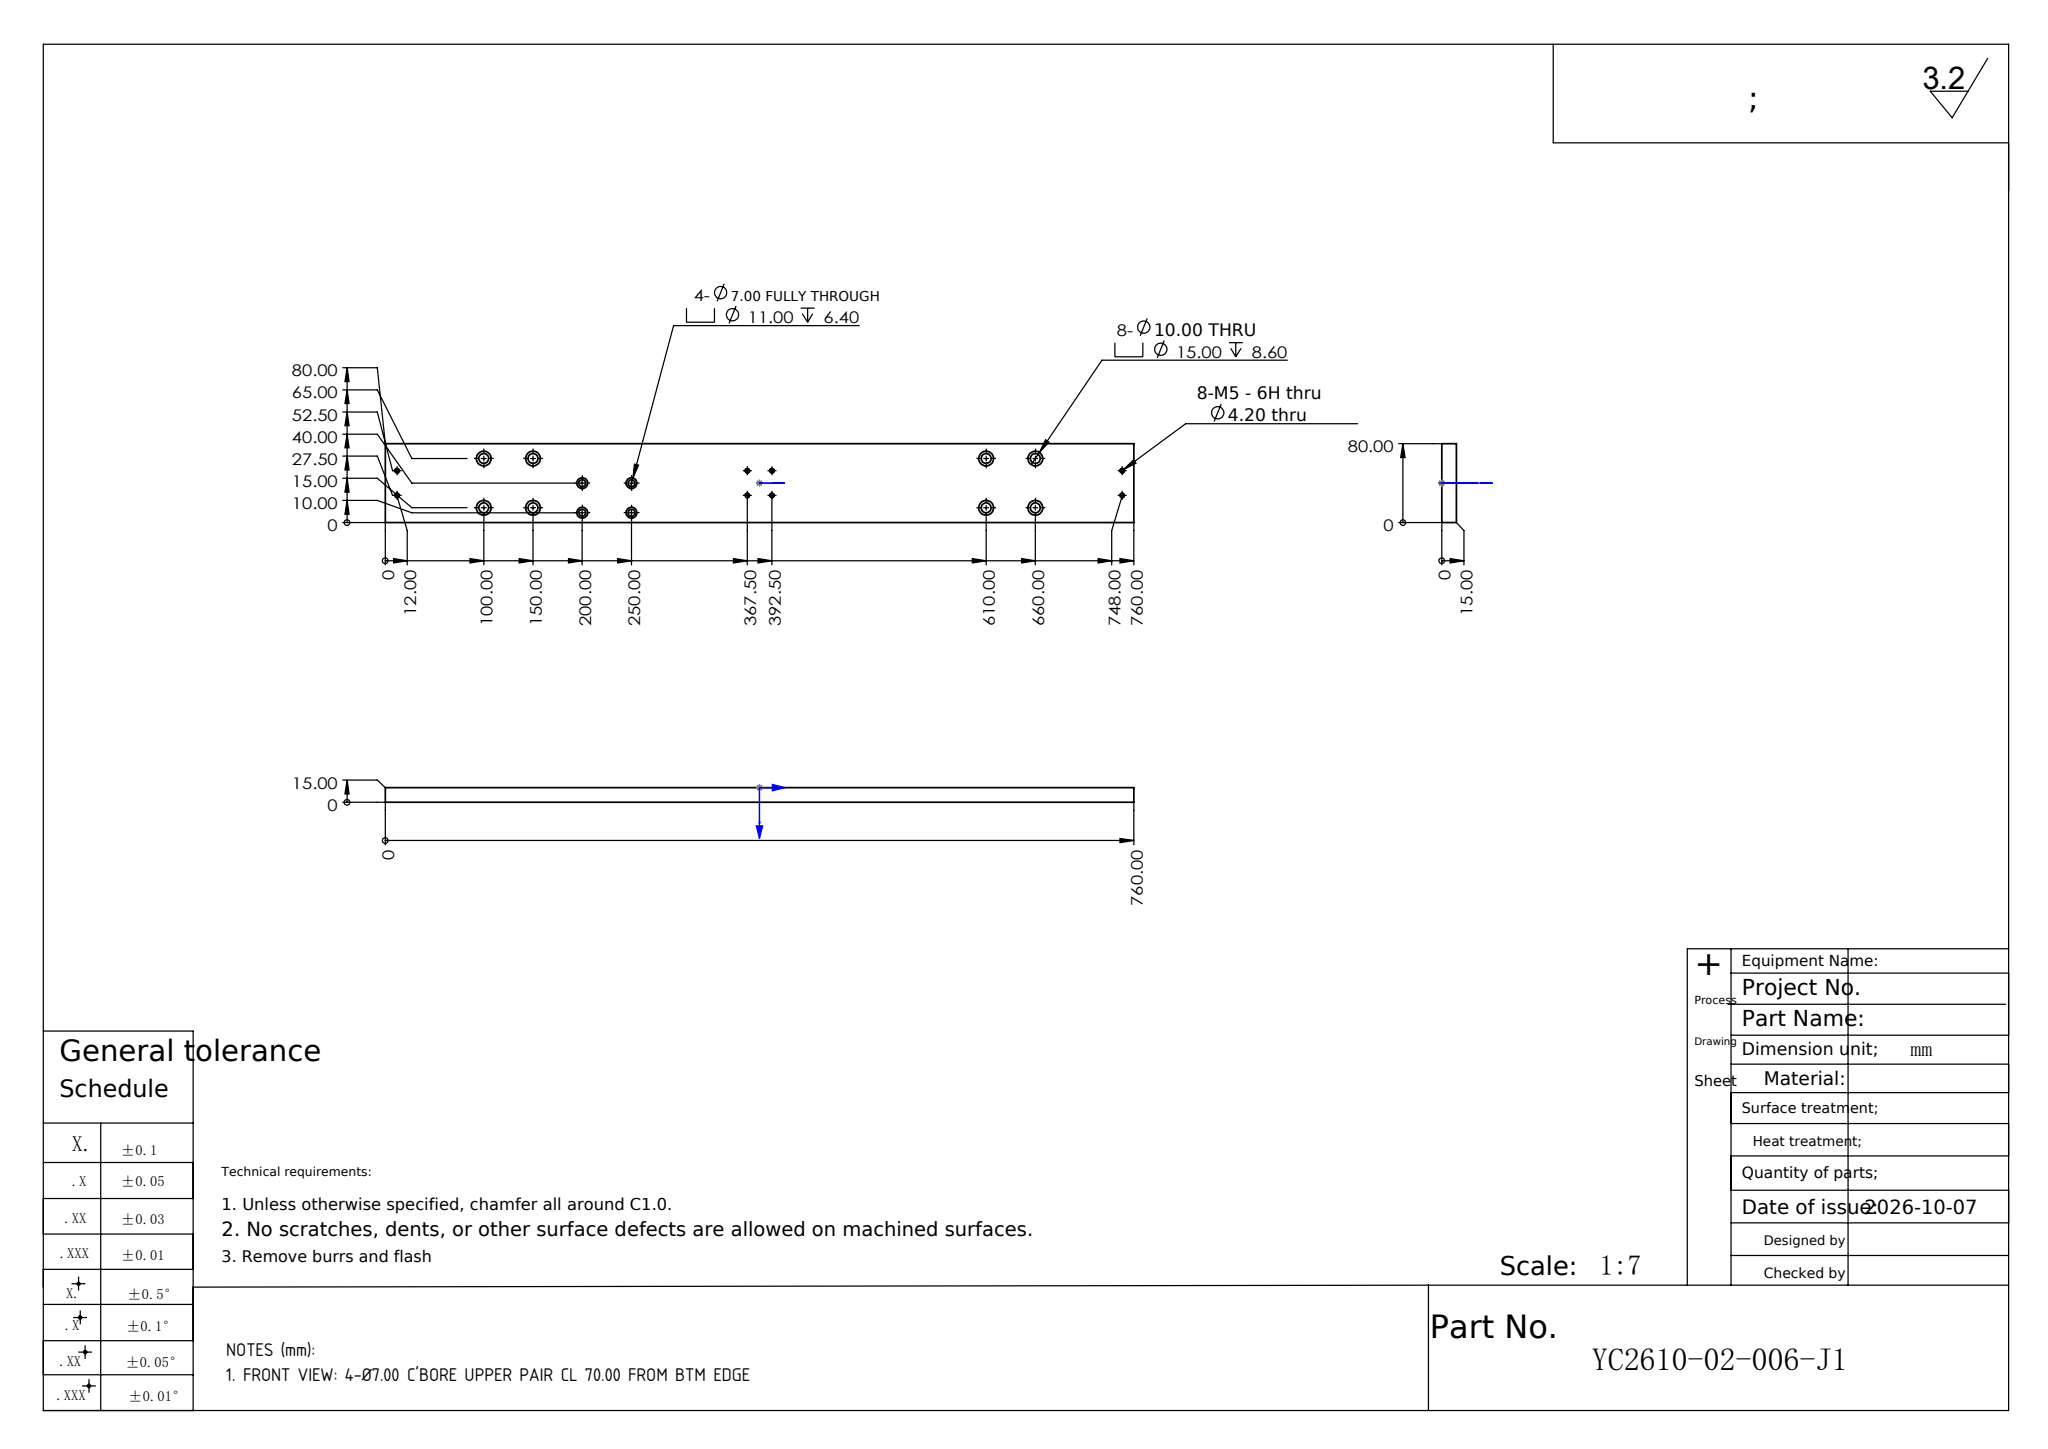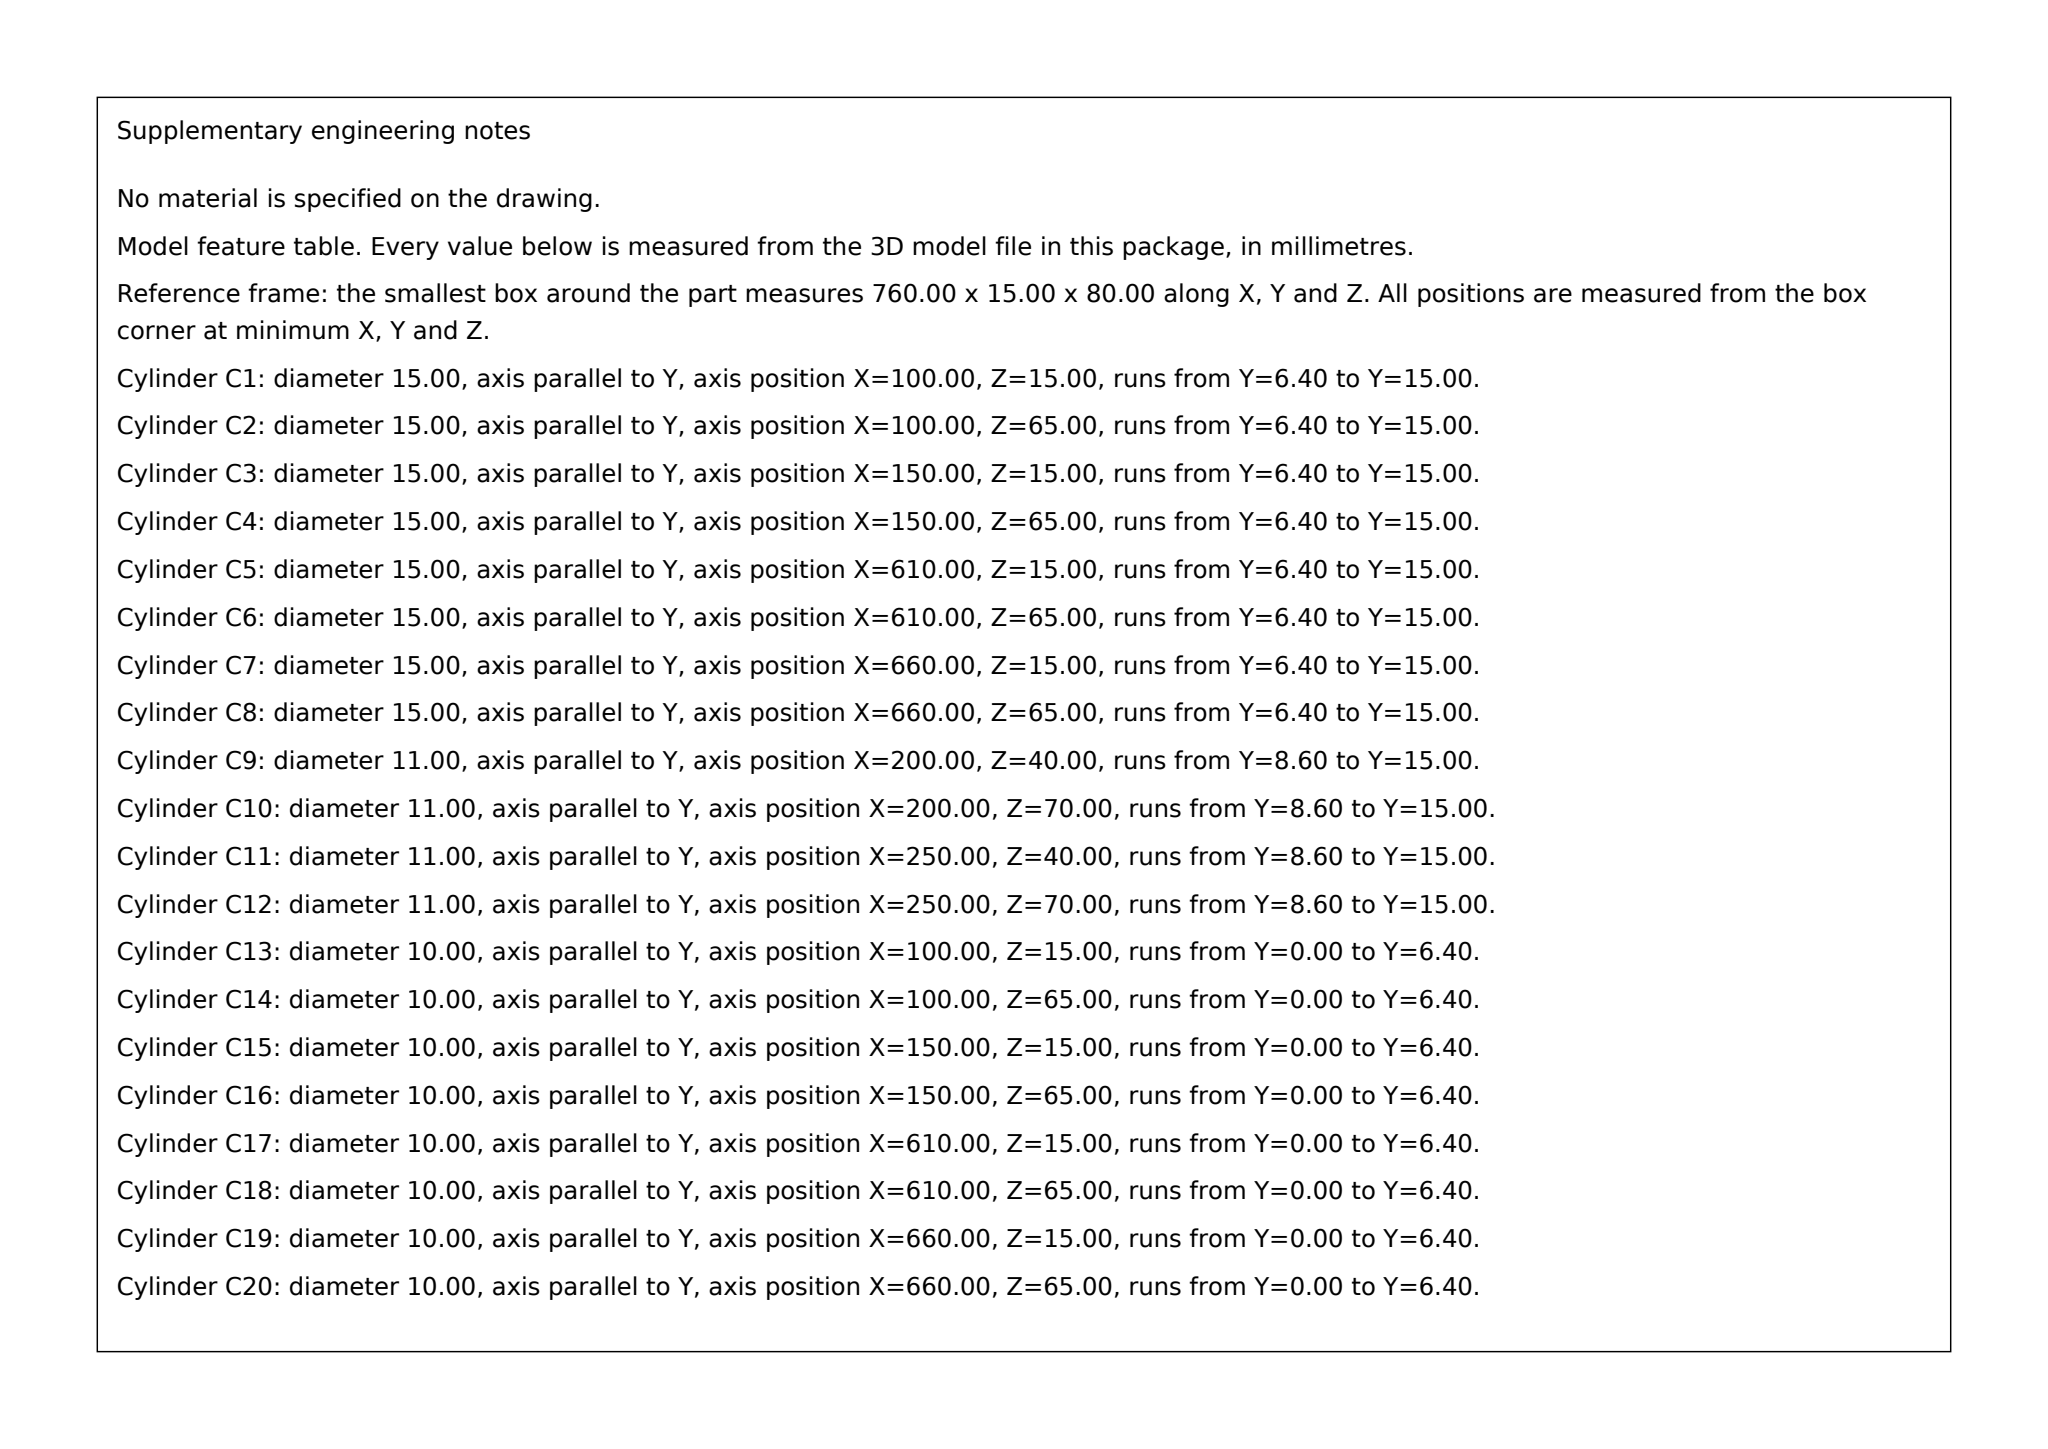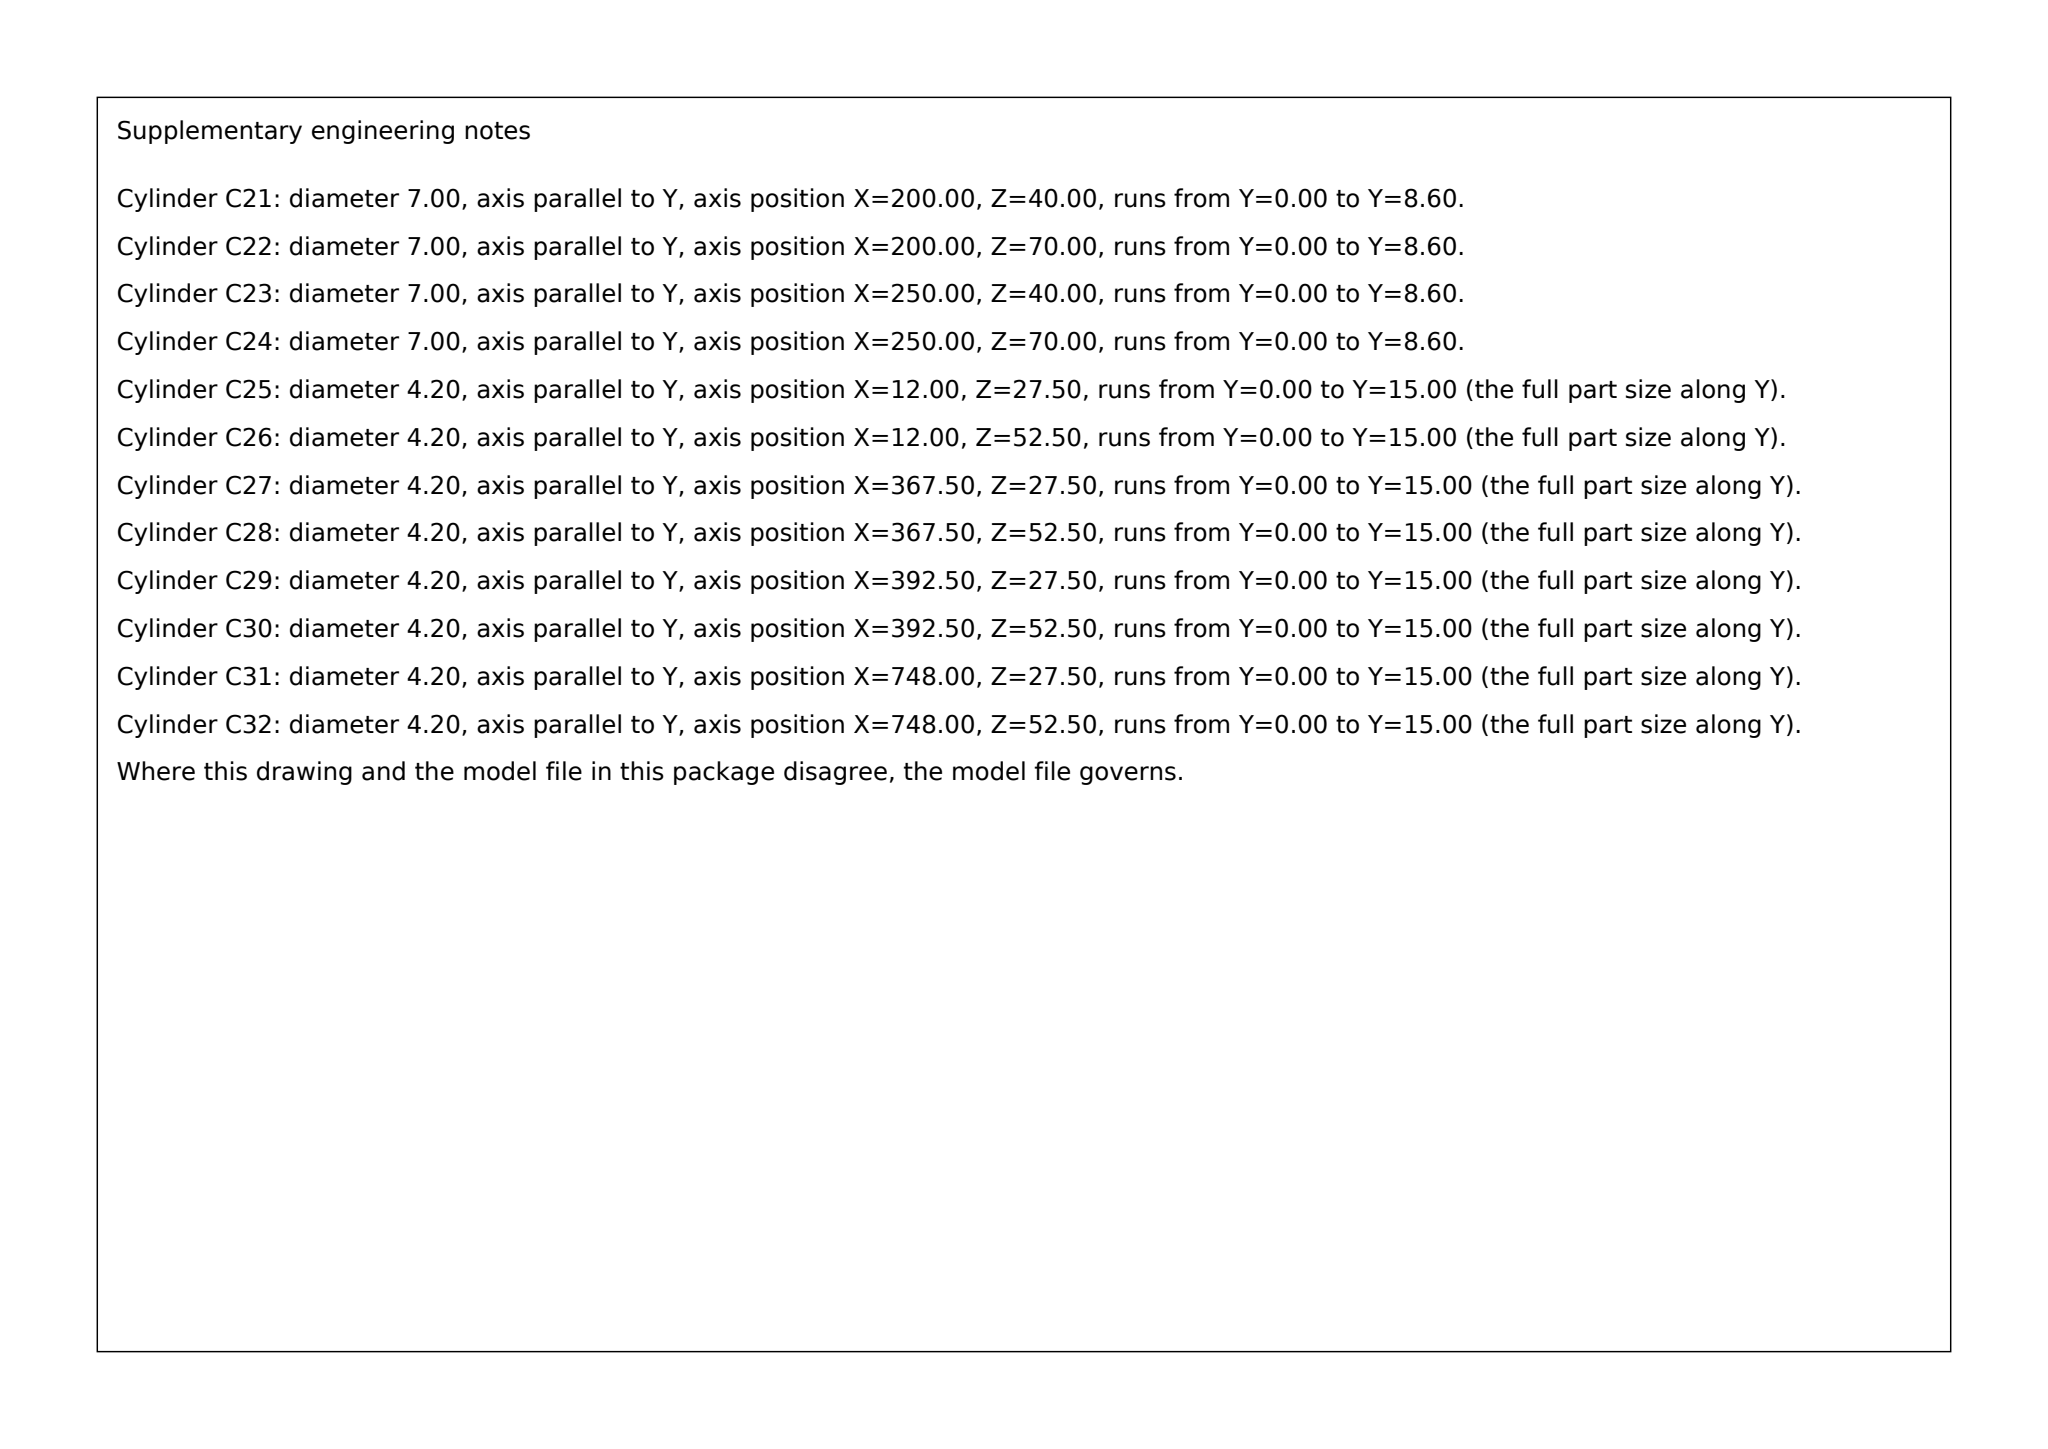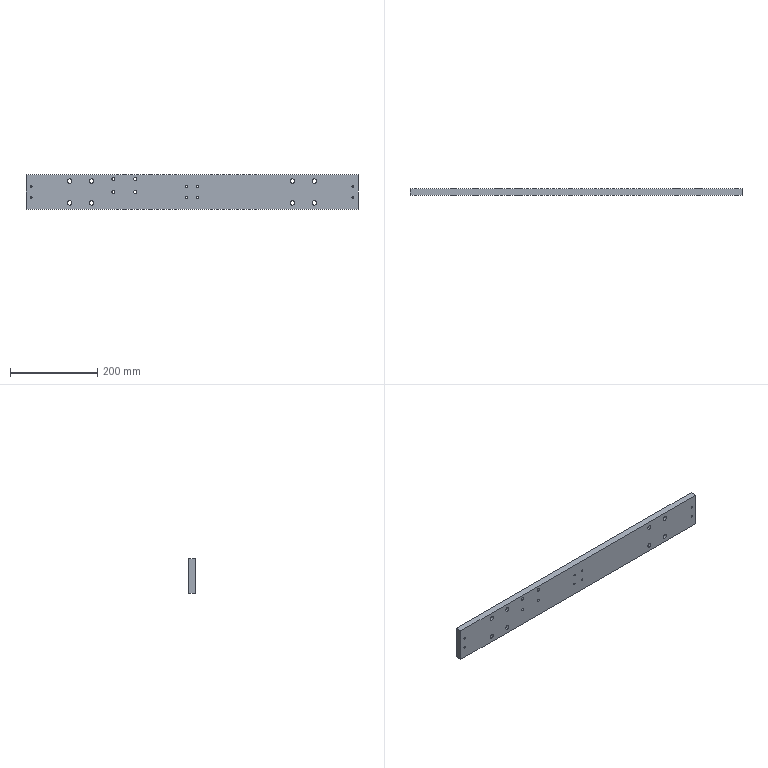Part | SolidWorks | mm | 1 solid | 82 faces | box 760 x 15 x 80 mm | volume 890402 mm3 | cylinder 64 | plane 18 | commonest cylinder face diameters 15 x16 10 x16 4.2 x16 11 x8 7 x8
Drawing notes:
FRONT VIEW: 4-Ø7.00 C'BORE UPPER PAIR CL 70.00 FROM BTM EDGE | from the solid: Ø7.0/Ø11.0 cyls at (x=200,z=70) and (x=250,z=70); bbox z=0..80
build123d program:
from build123d import *

# Parameters (mm, degrees)
SKETCH1_W                                       = 760
SKETCH1_H                                       = 80
BOSS_EXTRUDE1_DEPTH                             = 15
M5_TAPPED_HOLE1_D                               = 4.2
M6_HEX_SOCKET_HEAD_CAP_SCREW_CBORE1_D           = 7
M6_HEX_SOCKET_HEAD_CAP_SCREW_CBORE1_CBORE_D     = 11
M6_HEX_SOCKET_HEAD_CAP_SCREW_CBORE1_CBORE_DEPTH = 6.4
M8_HEX_SOCKET_HEAD_CAP_SCREW_CBORE1_D           = 10
M8_HEX_SOCKET_HEAD_CAP_SCREW_CBORE1_CBORE_D     = 15
M8_HEX_SOCKET_HEAD_CAP_SCREW_CBORE1_CBORE_DEPTH = 8.6


with BuildPart() as part:
    # Sketch1 → Boss-Extrude1 (new body)
    with BuildSketch(Plane(origin=(0, 0, 0), x_dir=(1, 0, 0), z_dir=(0, 1, 0))):
        Rectangle(SKETCH1_W, SKETCH1_H)
    extrude(amount=BOSS_EXTRUDE1_DEPTH)

    # M5 Tapped Hole1 (through all)
    with Locations(Plane(origin=(0, 15, 0), x_dir=(1, 0, 0), z_dir=(0, 1, 0))):
        with Locations((12.5, 12.5), (12.5, -12.5), (-12.5, -12.5), (-12.5, 12.5), (-368, 12.5), (-368, -12.5), (368, 12.5), (368, -12.5)):
            Hole(M5_TAPPED_HOLE1_D / 2)

    # M6 Hex Socket Head Cap Screw CBORE1 (through all)
    with Locations(Plane(origin=(0, 15, 0), x_dir=(1, 0, 0), z_dir=(0, 1, 0))):
        with Locations((-180, 0), (-130, 0), (-180, -30), (-130, -30)):
            CounterBoreHole(M6_HEX_SOCKET_HEAD_CAP_SCREW_CBORE1_D / 2, M6_HEX_SOCKET_HEAD_CAP_SCREW_CBORE1_CBORE_D / 2, M6_HEX_SOCKET_HEAD_CAP_SCREW_CBORE1_CBORE_DEPTH)

    # M8 Hex Socket Head Cap Screw CBORE1 (through all)
    with Locations(Plane(origin=(0, 15, 0), x_dir=(1, 0, 0), z_dir=(0, 1, 0))):
        with Locations((-280, 25), (-230, 25), (-280, -25), (-230, -25), (280, 25), (230, 25), (230, -25), (280, -25)):
            CounterBoreHole(M8_HEX_SOCKET_HEAD_CAP_SCREW_CBORE1_D / 2, M8_HEX_SOCKET_HEAD_CAP_SCREW_CBORE1_CBORE_D / 2, M8_HEX_SOCKET_HEAD_CAP_SCREW_CBORE1_CBORE_DEPTH)


solid = part.part